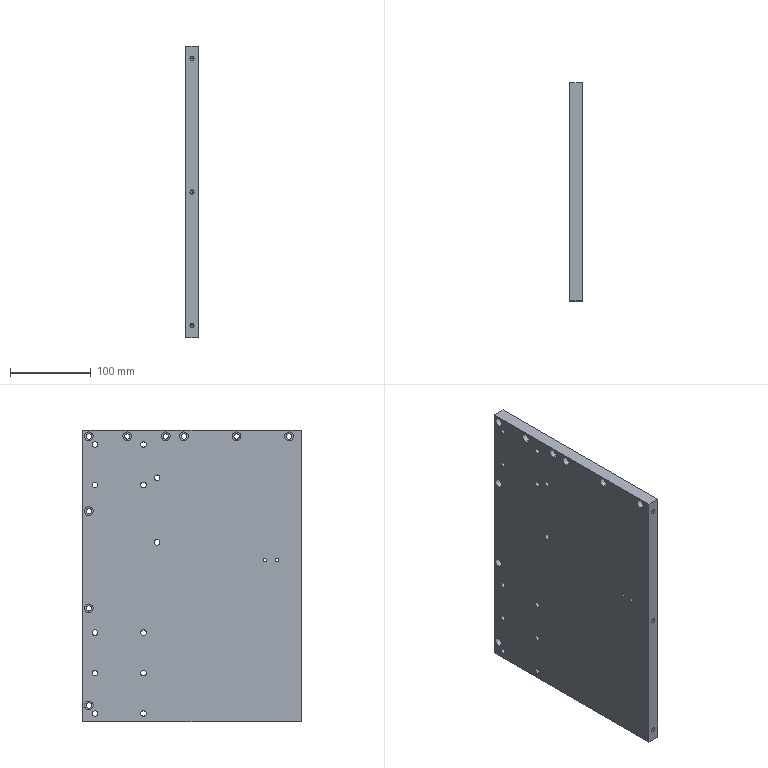Component | SolidWorks | SideFixingPlate3-1 | 1 solid | 105 faces | box 15 x 270 x 360 mm | volume 1440908 mm3 | cylinder 76 | plane 15 | cone 14 | commonest cylinder face diameters 6.8 x24 11 x18 6.6 x18 5 x12 4.2 x4 | material 1060 Alloy
build123d program:
from build123d import *

# Parameters (mm, degrees)
SKETCH1_W                                          = 360
SKETCH1_H                                          = 270
BOSS_EXTRUDE1_DEPTH                                = 15
HOLE_SIZE_ACCORDING_TO_TYPE_OF_HEXAGON_D           = 6.6
HOLE_SIZE_ACCORDING_TO_TYPE_OF_HEXAGON_CBORE_D     = 11
HOLE_SIZE_ACCORDING_TO_TYPE_OF_HEXAGON_CBORE_DEPTH = 6.8
HOLE_SIZE_ACCORDING_TO_TYPE_OF_HEX_2_D             = 6.6
HOLE_SIZE_ACCORDING_TO_TYPE_OF_HEX_2_CBORE_D       = 11
HOLE_SIZE_ACCORDING_TO_TYPE_OF_HEX_2_CBORE_DEPTH   = 6.8
M8_TAPPED_HOLE1_D                                  = 6.8
M6_TAPPED_HOLE1_D                                  = 5
M6_TAPPED_HOLE1_DEPTH                              = 15
M6_TAPPED_HOLE1_TIP                                = 1.502
M6_TAPPED_HOLE2_D                                  = 5
M6_TAPPED_HOLE2_DEPTH                              = 15
M6_TAPPED_HOLE2_TIP                                = 1.502
M8_TAPPED_HOLE2_D                                  = 6.8
M5_TAPPED_HOLE1_D                                  = 4.2


with BuildPart() as part:
    # Sketch1 → Boss-Extrude1 (new body)
    with BuildSketch(Plane.XY):
        with Locations((180, 0)):
            Rectangle(SKETCH1_W, SKETCH1_H)
    extrude(amount=BOSS_EXTRUDE1_DEPTH)

    # Hole Size _according to_ type of Hexagon (through all)
    with Locations(Plane.XY.offset(15)):
        with Locations((7.5, -32.5), (7.5, -80), (7.5, -127.5), (7.5, 120), (7.5, 55), (7.5, -10)):
            CounterBoreHole(HOLE_SIZE_ACCORDING_TO_TYPE_OF_HEXAGON_D / 2, HOLE_SIZE_ACCORDING_TO_TYPE_OF_HEXAGON_CBORE_D / 2, HOLE_SIZE_ACCORDING_TO_TYPE_OF_HEXAGON_CBORE_DEPTH)

    # Hole Size _according to_ type of Hex 2 (through all)
    with Locations(Plane.XY.offset(15)):
        with Locations((100, -127.5), (220, -127.5), (340, -127.5)):
            CounterBoreHole(HOLE_SIZE_ACCORDING_TO_TYPE_OF_HEX_2_D / 2, HOLE_SIZE_ACCORDING_TO_TYPE_OF_HEX_2_CBORE_D / 2, HOLE_SIZE_ACCORDING_TO_TYPE_OF_HEX_2_CBORE_DEPTH)

    # M8 Tapped Hole1 (through all)
    with Locations(Plane.XY.offset(15)):
        with Locations((58.5, -43), (138.5, -43)):
            Hole(M8_TAPPED_HOLE1_D / 2)

    # M6 Tapped Hole1
    with Locations(Plane(origin=(360, 0, 0), x_dir=(0, 0, -1), z_dir=(1, 0, 0))):
        with Locations((-7.5, 119.5), (-7.5, 7.5), (-7.5, -104.5)):
            Hole(M6_TAPPED_HOLE1_D / 2, depth=M6_TAPPED_HOLE1_DEPTH)
            with Locations((0, 0, -(M6_TAPPED_HOLE1_DEPTH + M6_TAPPED_HOLE1_TIP / 2))):  # 118° drill point
                Cone(0, M6_TAPPED_HOLE1_D / 2, M6_TAPPED_HOLE1_TIP, mode=Mode.SUBTRACT)

    # M6 Tapped Hole2
    with Locations(Plane(origin=(0, 135, 0), x_dir=(1, 0, 0), z_dir=(0, 1, 0))):
        with Locations((15, -7.5), (180, -7.5), (345, -7.5)):
            Hole(M6_TAPPED_HOLE2_D / 2, depth=M6_TAPPED_HOLE2_DEPTH)
            with Locations((0, 0, -(M6_TAPPED_HOLE2_DEPTH + M6_TAPPED_HOLE2_TIP / 2))):  # 118° drill point
                Cone(0, M6_TAPPED_HOLE2_D / 2, M6_TAPPED_HOLE2_TIP, mode=Mode.SUBTRACT)

    # M8 Tapped Hole2 (through all)
    with Locations(Plane.XY.offset(15)):
        with Locations((350, -60), (300, -60), (250, -60), (67.5, -120), (17.5, -120), (17.5, -60), (67.5, -60), (250, -120), (300, -120), (350, -120)):
            Hole(M8_TAPPED_HOLE2_D / 2)

    # M5 Tapped Hole1 (through all)
    with Locations(Plane(origin=(0, 0, 0), x_dir=(-1, 0, 0), z_dir=(0, 0, -1))):
        with Locations((-160.5, 105), (-160.5, 90)):
            Hole(M5_TAPPED_HOLE1_D / 2)


solid = part.part

# Placed as in the assembly
solid = solid.moved(Location((-129.666, 95.264, 197.5), (180, -90, 0)))